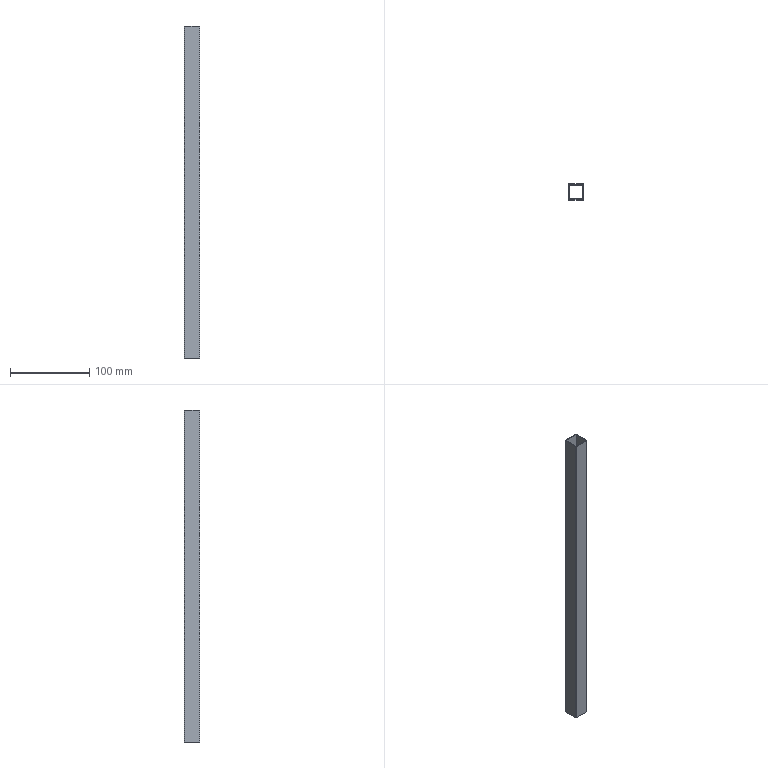Component | SolidWorks | Drawer_Rib-1 | 1 solid | 14 faces | box 20 x 20 x 420 mm | volume 37540 mm3 | plane 10 | cylinder 4 | commonest cylinder face diameters 2 x4
build123d program:
from build123d import *

# Parameters (mm, degrees)
SKETCH1_W           = 17.6
SKETCH1_H           = 17.6
BOSS_EXTRUDE1_DEPTH = 420


with BuildPart() as part:
    # Sketch1 → Boss-Extrude1 (new body)
    with BuildSketch(Plane(origin=(0, 0, 0), x_dir=(1, 0, 0), z_dir=(0, 1, 0))):
        with BuildLine():
            Line((-9, 10), (9, 10))
            ThreePointArc((9, 10), (9.707, 9.707), (10, 9))
            Line((10, 9), (10, -9))
            ThreePointArc((10, -9), (9.707, -9.707), (9, -10))
            Line((9, -10), (-9, -10))
            ThreePointArc((-9, -10), (-9.707, -9.707), (-10, -9))
            Line((-10, -9), (-10, 9))
            ThreePointArc((-10, 9), (-9.707, 9.707), (-9, 10))
        make_face()
        Rectangle(SKETCH1_W, SKETCH1_H, mode=Mode.SUBTRACT)
    extrude(amount=BOSS_EXTRUDE1_DEPTH)


solid = part.part

# Placed as in the assembly
solid = solid.moved(Location((8.5, 246, -100), (90, 0, 0)))
STEP:
#1=COLOUR_RGB('',0.7922,0.8196,0.9333);
#2=FILL_AREA_STYLE_COLOUR('',#1);
#3=FILL_AREA_STYLE('',(#2));
#4=SURFACE_STYLE_FILL_AREA(#3);
#5=SURFACE_SIDE_STYLE('',(#4));
#6=SURFACE_STYLE_USAGE(.BOTH.,#5);
#7=PRESENTATION_STYLE_ASSIGNMENT((#6));
#8=CARTESIAN_POINT('',(-0.01969,9.291,-3.937));
#9=VERTEX_POINT('',#8);
#10=CARTESIAN_POINT('',(-0.05906,9.331,-3.937));
#11=VERTEX_POINT('',#10);
#12=CARTESIAN_POINT('',(-0.01969,9.331,-3.937));
#13=DIRECTION('',(0.,-0.,-1.));
#14=DIRECTION('',(-1.,0.,0.));
#15=AXIS2_PLACEMENT_3D('',#12,#13,#14);
#16=CIRCLE('',#15,0.03937);
#17=EDGE_CURVE('',#9,#11,#16,.T.);
#18=ORIENTED_EDGE('',*,*,#17,.T.);
#19=CARTESIAN_POINT('',(-0.05906,10.039,-3.937));
#20=VERTEX_POINT('',#19);
#21=CARTESIAN_POINT('',(-0.05906,9.331,-3.937));
#22=DIRECTION('',(-0.,1.,-0.));
#23=VECTOR('',#22,39.37);
#24=LINE('',#21,#23);
#25=EDGE_CURVE('',#11,#20,#24,.T.);
#26=ORIENTED_EDGE('',*,*,#25,.T.);
#27=CARTESIAN_POINT('',(-0.01969,10.079,-3.937));
#28=VERTEX_POINT('',#27);
#29=CARTESIAN_POINT('',(-0.01969,10.039,-3.937));
#30=DIRECTION('',(0.,-0.,-1.));
#31=DIRECTION('',(1.,0.,0.));
#32=AXIS2_PLACEMENT_3D('',#29,#30,#31);
#33=CIRCLE('',#32,0.03937);
#34=EDGE_CURVE('',#20,#28,#33,.T.);
#35=ORIENTED_EDGE('',*,*,#34,.T.);
#36=CARTESIAN_POINT('',(0.689,10.079,-3.937));
#37=VERTEX_POINT('',#36);
#38=CARTESIAN_POINT('',(0.689,10.079,-3.937));
#39=DIRECTION('',(1.,-0.,0.));
#40=VECTOR('',#39,39.37);
#41=LINE('',#38,#40);
#42=EDGE_CURVE('',#28,#37,#41,.T.);
#43=ORIENTED_EDGE('',*,*,#42,.T.);
#44=CARTESIAN_POINT('',(0.7283,10.039,-3.937));
#45=VERTEX_POINT('',#44);
#46=CARTESIAN_POINT('',(0.689,10.039,-3.937));
#47=DIRECTION('',(0.,-0.,-1.));
#48=DIRECTION('',(-1.,0.,0.));
#49=AXIS2_PLACEMENT_3D('',#46,#47,#48);
#50=CIRCLE('',#49,0.03937);
#51=EDGE_CURVE('',#37,#45,#50,.T.);
#52=ORIENTED_EDGE('',*,*,#51,.T.);
#53=CARTESIAN_POINT('',(0.7283,9.331,-3.937));
#54=VERTEX_POINT('',#53);
#55=CARTESIAN_POINT('',(0.7283,9.331,-3.937));
#56=DIRECTION('',(0.,-1.,0.));
#57=VECTOR('',#56,39.37);
#58=LINE('',#55,#57);
#59=EDGE_CURVE('',#45,#54,#58,.T.);
#60=ORIENTED_EDGE('',*,*,#59,.T.);
#61=CARTESIAN_POINT('',(0.689,9.291,-3.937));
#62=VERTEX_POINT('',#61);
#63=CARTESIAN_POINT('',(0.689,9.331,-3.937));
#64=DIRECTION('',(0.,-0.,-1.));
#65=DIRECTION('',(-1.,0.,0.));
#66=AXIS2_PLACEMENT_3D('',#63,#64,#65);
#67=CIRCLE('',#66,0.03937);
#68=EDGE_CURVE('',#54,#62,#67,.T.);
#69=ORIENTED_EDGE('',*,*,#68,.T.);
#70=CARTESIAN_POINT('',(0.689,9.291,-3.937));
#71=DIRECTION('',(-1.,0.,-0.));
#72=VECTOR('',#71,39.37);
#73=LINE('',#70,#72);
#74=EDGE_CURVE('',#62,#9,#73,.T.);
#75=ORIENTED_EDGE('',*,*,#74,.T.);
#76=EDGE_LOOP('',(#18,#26,#35,#43,#52,#60,#69,#75));
#77=FACE_OUTER_BOUND('',#76,.T.);
#78=CARTESIAN_POINT('',(0.6811,9.339,-3.937));
#79=VERTEX_POINT('',#78);
#80=CARTESIAN_POINT('',(-0.01181,9.339,-3.937));
#81=VERTEX_POINT('',#80);
#82=CARTESIAN_POINT('',(0.6811,9.339,-3.937));
#83=DIRECTION('',(-1.,-0.,-0.));
#84=VECTOR('',#83,39.37);
#85=LINE('',#82,#84);
#86=EDGE_CURVE('',#79,#81,#85,.T.);
#87=ORIENTED_EDGE('',*,*,#86,.F.);
#88=CARTESIAN_POINT('',(0.6811,10.031,-3.937));
#89=VERTEX_POINT('',#88);
#90=CARTESIAN_POINT('',(0.6811,9.339,-3.937));
#91=DIRECTION('',(0.,-1.,0.));
#92=VECTOR('',#91,39.37);
#93=LINE('',#90,#92);
#94=EDGE_CURVE('',#89,#79,#93,.T.);
#95=ORIENTED_EDGE('',*,*,#94,.F.);
#96=CARTESIAN_POINT('',(-0.01181,10.031,-3.937));
#97=VERTEX_POINT('',#96);
#98=CARTESIAN_POINT('',(0.6811,10.031,-3.937));
#99=DIRECTION('',(1.,0.,0.));
#100=VECTOR('',#99,39.37);
#101=LINE('',#98,#100);
#102=EDGE_CURVE('',#97,#89,#101,.T.);
#103=ORIENTED_EDGE('',*,*,#102,.F.);
#104=CARTESIAN_POINT('',(-0.01181,9.339,-3.937));
#105=DIRECTION('',(-0.,1.,-0.));
#106=VECTOR('',#105,39.37);
#107=LINE('',#104,#106);
#108=EDGE_CURVE('',#81,#97,#107,.T.);
#109=ORIENTED_EDGE('',*,*,#108,.F.);
#110=EDGE_LOOP('',(#87,#95,#103,#109));
#111=FACE_BOUND('',#110,.T.);
#112=CARTESIAN_POINT('',(-0.01969,9.331,-3.937));
#113=DIRECTION('',(0.,-0.,-1.));
#114=DIRECTION('',(-1.,-0.,-0.));
#115=AXIS2_PLACEMENT_3D('',#112,#113,#114);
#116=PLANE('',#115);
#117=ADVANCED_FACE('',(#77,#111),#116,.T.);
#118=CARTESIAN_POINT('',(-0.01969,9.291,12.598));
#119=VERTEX_POINT('',#118);
#120=CARTESIAN_POINT('',(-0.05906,9.331,12.598));
#121=VERTEX_POINT('',#120);
#122=CARTESIAN_POINT('',(-0.01969,9.331,12.598));
#123=DIRECTION('',(0.,-0.,-1.));
#124=DIRECTION('',(-1.,0.,0.));
#125=AXIS2_PLACEMENT_3D('',#122,#123,#124);
#126=CIRCLE('',#125,0.03937);
#127=EDGE_CURVE('',#119,#121,#126,.T.);
#128=ORIENTED_EDGE('',*,*,#127,.F.);
#129=CARTESIAN_POINT('',(0.689,9.291,12.598));
#130=VERTEX_POINT('',#129);
#131=CARTESIAN_POINT('',(0.689,9.291,12.598));
#132=DIRECTION('',(-1.,0.,-0.));
#133=VECTOR('',#132,39.37);
#134=LINE('',#131,#133);
#135=EDGE_CURVE('',#130,#119,#134,.T.);
#136=ORIENTED_EDGE('',*,*,#135,.F.);
#137=CARTESIAN_POINT('',(0.7283,9.331,12.598));
#138=VERTEX_POINT('',#137);
#139=CARTESIAN_POINT('',(0.689,9.331,12.598));
#140=DIRECTION('',(0.,-0.,-1.));
#141=DIRECTION('',(-1.,0.,0.));
#142=AXIS2_PLACEMENT_3D('',#139,#140,#141);
#143=CIRCLE('',#142,0.03937);
#144=EDGE_CURVE('',#138,#130,#143,.T.);
#145=ORIENTED_EDGE('',*,*,#144,.F.);
#146=CARTESIAN_POINT('',(0.7283,10.039,12.598));
#147=VERTEX_POINT('',#146);
#148=CARTESIAN_POINT('',(0.7283,9.331,12.598));
#149=DIRECTION('',(0.,-1.,0.));
#150=VECTOR('',#149,39.37);
#151=LINE('',#148,#150);
#152=EDGE_CURVE('',#147,#138,#151,.T.);
#153=ORIENTED_EDGE('',*,*,#152,.F.);
#154=CARTESIAN_POINT('',(0.689,10.079,12.598));
#155=VERTEX_POINT('',#154);
#156=CARTESIAN_POINT('',(0.689,10.039,12.598));
#157=DIRECTION('',(0.,-0.,-1.));
#158=DIRECTION('',(-1.,0.,0.));
#159=AXIS2_PLACEMENT_3D('',#156,#157,#158);
#160=CIRCLE('',#159,0.03937);
#161=EDGE_CURVE('',#155,#147,#160,.T.);
#162=ORIENTED_EDGE('',*,*,#161,.F.);
#163=CARTESIAN_POINT('',(-0.01969,10.079,12.598));
#164=VERTEX_POINT('',#163);
#165=CARTESIAN_POINT('',(0.689,10.079,12.598));
#166=DIRECTION('',(1.,-0.,0.));
#167=VECTOR('',#166,39.37);
#168=LINE('',#165,#167);
#169=EDGE_CURVE('',#164,#155,#168,.T.);
#170=ORIENTED_EDGE('',*,*,#169,.F.);
#171=CARTESIAN_POINT('',(-0.05906,10.039,12.598));
#172=VERTEX_POINT('',#171);
#173=CARTESIAN_POINT('',(-0.01969,10.039,12.598));
#174=DIRECTION('',(0.,-0.,-1.));
#175=DIRECTION('',(1.,0.,0.));
#176=AXIS2_PLACEMENT_3D('',#173,#174,#175);
#177=CIRCLE('',#176,0.03937);
#178=EDGE_CURVE('',#172,#164,#177,.T.);
#179=ORIENTED_EDGE('',*,*,#178,.F.);
#180=CARTESIAN_POINT('',(-0.05906,9.331,12.598));
#181=DIRECTION('',(-0.,1.,-0.));
#182=VECTOR('',#181,39.37);
#183=LINE('',#180,#182);
#184=EDGE_CURVE('',#121,#172,#183,.T.);
#185=ORIENTED_EDGE('',*,*,#184,.F.);
#186=EDGE_LOOP('',(#128,#136,#145,#153,#162,#170,#179,#185));
#187=FACE_OUTER_BOUND('',#186,.T.);
#188=CARTESIAN_POINT('',(0.6811,10.031,12.598));
#189=VERTEX_POINT('',#188);
#190=CARTESIAN_POINT('',(0.6811,9.339,12.598));
#191=VERTEX_POINT('',#190);
#192=CARTESIAN_POINT('',(0.6811,9.339,12.598));
#193=DIRECTION('',(0.,-1.,0.));
#194=VECTOR('',#193,39.37);
#195=LINE('',#192,#194);
#196=EDGE_CURVE('',#189,#191,#195,.T.);
#197=ORIENTED_EDGE('',*,*,#196,.T.);
#198=CARTESIAN_POINT('',(-0.01181,9.339,12.598));
#199=VERTEX_POINT('',#198);
#200=CARTESIAN_POINT('',(0.6811,9.339,12.598));
#201=DIRECTION('',(-1.,-0.,-0.));
#202=VECTOR('',#201,39.37);
#203=LINE('',#200,#202);
#204=EDGE_CURVE('',#191,#199,#203,.T.);
#205=ORIENTED_EDGE('',*,*,#204,.T.);
#206=CARTESIAN_POINT('',(-0.01181,10.031,12.598));
#207=VERTEX_POINT('',#206);
#208=CARTESIAN_POINT('',(-0.01181,9.339,12.598));
#209=DIRECTION('',(-0.,1.,-0.));
#210=VECTOR('',#209,39.37);
#211=LINE('',#208,#210);
#212=EDGE_CURVE('',#199,#207,#211,.T.);
#213=ORIENTED_EDGE('',*,*,#212,.T.);
#214=CARTESIAN_POINT('',(0.6811,10.031,12.598));
#215=DIRECTION('',(1.,0.,0.));
#216=VECTOR('',#215,39.37);
#217=LINE('',#214,#216);
#218=EDGE_CURVE('',#207,#189,#217,.T.);
#219=ORIENTED_EDGE('',*,*,#218,.T.);
#220=EDGE_LOOP('',(#197,#205,#213,#219));
#221=FACE_BOUND('',#220,.T.);
#222=CARTESIAN_POINT('',(-0.01969,9.331,12.598));
#223=DIRECTION('',(0.,-0.,-1.));
#224=DIRECTION('',(-1.,-0.,-0.));
#225=AXIS2_PLACEMENT_3D('',#222,#223,#224);
#226=PLANE('',#225);
#227=ADVANCED_FACE('',(#187,#221),#226,.F.);
#228=ORIENTED_EDGE('',*,*,#127,.T.);
#229=CARTESIAN_POINT('',(-0.05906,9.331,-3.937));
#230=DIRECTION('',(-0.,0.,1.));
#231=VECTOR('',#230,39.37);
#232=LINE('',#229,#231);
#233=EDGE_CURVE('',#11,#121,#232,.T.);
#234=ORIENTED_EDGE('',*,*,#233,.F.);
#235=ORIENTED_EDGE('',*,*,#17,.F.);
#236=CARTESIAN_POINT('',(-0.01969,9.291,-3.937));
#237=DIRECTION('',(-0.,0.,1.));
#238=VECTOR('',#237,39.37);
#239=LINE('',#236,#238);
#240=EDGE_CURVE('',#9,#119,#239,.T.);
#241=ORIENTED_EDGE('',*,*,#240,.T.);
#242=EDGE_LOOP('',(#228,#234,#235,#241));
#243=FACE_OUTER_BOUND('',#242,.T.);
#244=CARTESIAN_POINT('',(-0.01969,9.331,-3.937));
#245=DIRECTION('',(-0.,0.,1.));
#246=DIRECTION('',(1.,0.,0.));
#247=AXIS2_PLACEMENT_3D('',#244,#245,#246);
#248=CYLINDRICAL_SURFACE('',#247,0.03937);
#249=ADVANCED_FACE('',(#243),#248,.T.);
#250=ORIENTED_EDGE('',*,*,#184,.T.);
#251=CARTESIAN_POINT('',(-0.05906,10.039,-3.937));
#252=DIRECTION('',(-0.,0.,1.));
#253=VECTOR('',#252,39.37);
#254=LINE('',#251,#253);
#255=EDGE_CURVE('',#20,#172,#254,.T.);
#256=ORIENTED_EDGE('',*,*,#255,.F.);
#257=ORIENTED_EDGE('',*,*,#25,.F.);
#258=ORIENTED_EDGE('',*,*,#233,.T.);
#259=EDGE_LOOP('',(#250,#256,#257,#258));
#260=FACE_OUTER_BOUND('',#259,.T.);
#261=CARTESIAN_POINT('',(-0.05906,9.331,-3.937));
#262=DIRECTION('',(1.,0.,0.));
#263=DIRECTION('',(0.,-1.,0.));
#264=AXIS2_PLACEMENT_3D('',#261,#262,#263);
#265=PLANE('',#264);
#266=ADVANCED_FACE('',(#260),#265,.F.);
#267=ORIENTED_EDGE('',*,*,#178,.T.);
#268=CARTESIAN_POINT('',(-0.01969,10.079,-3.937));
#269=DIRECTION('',(-0.,0.,1.));
#270=VECTOR('',#269,39.37);
#271=LINE('',#268,#270);
#272=EDGE_CURVE('',#28,#164,#271,.T.);
#273=ORIENTED_EDGE('',*,*,#272,.F.);
#274=ORIENTED_EDGE('',*,*,#34,.F.);
#275=ORIENTED_EDGE('',*,*,#255,.T.);
#276=EDGE_LOOP('',(#267,#273,#274,#275));
#277=FACE_OUTER_BOUND('',#276,.T.);
#278=CARTESIAN_POINT('',(-0.01969,10.039,-3.937));
#279=DIRECTION('',(-0.,0.,1.));
#280=DIRECTION('',(1.,0.,0.));
#281=AXIS2_PLACEMENT_3D('',#278,#279,#280);
#282=CYLINDRICAL_SURFACE('',#281,0.03937);
#283=ADVANCED_FACE('',(#277),#282,.T.);
#284=ORIENTED_EDGE('',*,*,#169,.T.);
#285=CARTESIAN_POINT('',(0.689,10.079,-3.937));
#286=DIRECTION('',(-0.,0.,1.));
#287=VECTOR('',#286,39.37);
#288=LINE('',#285,#287);
#289=EDGE_CURVE('',#37,#155,#288,.T.);
#290=ORIENTED_EDGE('',*,*,#289,.F.);
#291=ORIENTED_EDGE('',*,*,#42,.F.);
#292=ORIENTED_EDGE('',*,*,#272,.T.);
#293=EDGE_LOOP('',(#284,#290,#291,#292));
#294=FACE_OUTER_BOUND('',#293,.T.);
#295=CARTESIAN_POINT('',(0.689,10.079,-3.937));
#296=DIRECTION('',(-0.,-1.,0.));
#297=DIRECTION('',(-1.,0.,-0.));
#298=AXIS2_PLACEMENT_3D('',#295,#296,#297);
#299=PLANE('',#298);
#300=ADVANCED_FACE('',(#294),#299,.F.);
#301=ORIENTED_EDGE('',*,*,#161,.T.);
#302=CARTESIAN_POINT('',(0.7283,10.039,-3.937));
#303=DIRECTION('',(-0.,0.,1.));
#304=VECTOR('',#303,39.37);
#305=LINE('',#302,#304);
#306=EDGE_CURVE('',#45,#147,#305,.T.);
#307=ORIENTED_EDGE('',*,*,#306,.F.);
#308=ORIENTED_EDGE('',*,*,#51,.F.);
#309=ORIENTED_EDGE('',*,*,#289,.T.);
#310=EDGE_LOOP('',(#301,#307,#308,#309));
#311=FACE_OUTER_BOUND('',#310,.T.);
#312=CARTESIAN_POINT('',(0.689,10.039,-3.937));
#313=DIRECTION('',(-0.,0.,1.));
#314=DIRECTION('',(1.,0.,0.));
#315=AXIS2_PLACEMENT_3D('',#312,#313,#314);
#316=CYLINDRICAL_SURFACE('',#315,0.03937);
#317=ADVANCED_FACE('',(#311),#316,.T.);
#318=ORIENTED_EDGE('',*,*,#152,.T.);
#319=CARTESIAN_POINT('',(0.7283,9.331,-3.937));
#320=DIRECTION('',(-0.,0.,1.));
#321=VECTOR('',#320,39.37);
#322=LINE('',#319,#321);
#323=EDGE_CURVE('',#54,#138,#322,.T.);
#324=ORIENTED_EDGE('',*,*,#323,.F.);
#325=ORIENTED_EDGE('',*,*,#59,.F.);
#326=ORIENTED_EDGE('',*,*,#306,.T.);
#327=EDGE_LOOP('',(#318,#324,#325,#326));
#328=FACE_OUTER_BOUND('',#327,.T.);
#329=CARTESIAN_POINT('',(0.7283,9.331,-3.937));
#330=DIRECTION('',(-1.,-0.,-0.));
#331=DIRECTION('',(-0.,1.,-0.));
#332=AXIS2_PLACEMENT_3D('',#329,#330,#331);
#333=PLANE('',#332);
#334=ADVANCED_FACE('',(#328),#333,.F.);
#335=ORIENTED_EDGE('',*,*,#144,.T.);
#336=CARTESIAN_POINT('',(0.689,9.291,-3.937));
#337=DIRECTION('',(-0.,0.,1.));
#338=VECTOR('',#337,39.37);
#339=LINE('',#336,#338);
#340=EDGE_CURVE('',#62,#130,#339,.T.);
#341=ORIENTED_EDGE('',*,*,#340,.F.);
#342=ORIENTED_EDGE('',*,*,#68,.F.);
#343=ORIENTED_EDGE('',*,*,#323,.T.);
#344=EDGE_LOOP('',(#335,#341,#342,#343));
#345=FACE_OUTER_BOUND('',#344,.T.);
#346=CARTESIAN_POINT('',(0.689,9.331,-3.937));
#347=DIRECTION('',(-0.,0.,1.));
#348=DIRECTION('',(1.,0.,0.));
#349=AXIS2_PLACEMENT_3D('',#346,#347,#348);
#350=CYLINDRICAL_SURFACE('',#349,0.03937);
#351=ADVANCED_FACE('',(#345),#350,.T.);
#352=ORIENTED_EDGE('',*,*,#135,.T.);
#353=ORIENTED_EDGE('',*,*,#240,.F.);
#354=ORIENTED_EDGE('',*,*,#74,.F.);
#355=ORIENTED_EDGE('',*,*,#340,.T.);
#356=EDGE_LOOP('',(#352,#353,#354,#355));
#357=FACE_OUTER_BOUND('',#356,.T.);
#358=CARTESIAN_POINT('',(0.689,9.291,-3.937));
#359=DIRECTION('',(0.,1.,-0.));
#360=DIRECTION('',(1.,-0.,0.));
#361=AXIS2_PLACEMENT_3D('',#358,#359,#360);
#362=PLANE('',#361);
#363=ADVANCED_FACE('',(#357),#362,.F.);
#364=ORIENTED_EDGE('',*,*,#196,.F.);
#365=CARTESIAN_POINT('',(0.6811,10.031,-3.937));
#366=DIRECTION('',(-0.,0.,1.));
#367=VECTOR('',#366,39.37);
#368=LINE('',#365,#367);
#369=EDGE_CURVE('',#89,#189,#368,.T.);
#370=ORIENTED_EDGE('',*,*,#369,.F.);
#371=ORIENTED_EDGE('',*,*,#94,.T.);
#372=CARTESIAN_POINT('',(0.6811,9.339,-3.937));
#373=DIRECTION('',(-0.,0.,1.));
#374=VECTOR('',#373,39.37);
#375=LINE('',#372,#374);
#376=EDGE_CURVE('',#79,#191,#375,.T.);
#377=ORIENTED_EDGE('',*,*,#376,.T.);
#378=EDGE_LOOP('',(#364,#370,#371,#377));
#379=FACE_OUTER_BOUND('',#378,.T.);
#380=CARTESIAN_POINT('',(0.6811,9.339,-3.937));
#381=DIRECTION('',(-1.,-0.,-0.));
#382=DIRECTION('',(-0.,1.,-0.));
#383=AXIS2_PLACEMENT_3D('',#380,#381,#382);
#384=PLANE('',#383);
#385=ADVANCED_FACE('',(#379),#384,.T.);
#386=ORIENTED_EDGE('',*,*,#204,.F.);
#387=ORIENTED_EDGE('',*,*,#376,.F.);
#388=ORIENTED_EDGE('',*,*,#86,.T.);
#389=CARTESIAN_POINT('',(-0.01181,9.339,-3.937));
#390=DIRECTION('',(-0.,0.,1.));
#391=VECTOR('',#390,39.37);
#392=LINE('',#389,#391);
#393=EDGE_CURVE('',#81,#199,#392,.T.);
#394=ORIENTED_EDGE('',*,*,#393,.T.);
#395=EDGE_LOOP('',(#386,#387,#388,#394));
#396=FACE_OUTER_BOUND('',#395,.T.);
#397=CARTESIAN_POINT('',(0.6811,9.339,-3.937));
#398=DIRECTION('',(-0.,1.,-0.));
#399=DIRECTION('',(1.,0.,0.));
#400=AXIS2_PLACEMENT_3D('',#397,#398,#399);
#401=PLANE('',#400);
#402=ADVANCED_FACE('',(#396),#401,.T.);
#403=ORIENTED_EDGE('',*,*,#212,.F.);
#404=ORIENTED_EDGE('',*,*,#393,.F.);
#405=ORIENTED_EDGE('',*,*,#108,.T.);
#406=CARTESIAN_POINT('',(-0.01181,10.031,-3.937));
#407=DIRECTION('',(-0.,0.,1.));
#408=VECTOR('',#407,39.37);
#409=LINE('',#406,#408);
#410=EDGE_CURVE('',#97,#207,#409,.T.);
#411=ORIENTED_EDGE('',*,*,#410,.T.);
#412=EDGE_LOOP('',(#403,#404,#405,#411));
#413=FACE_OUTER_BOUND('',#412,.T.);
#414=CARTESIAN_POINT('',(-0.01181,9.339,-3.937));
#415=DIRECTION('',(1.,0.,0.));
#416=DIRECTION('',(0.,-1.,0.));
#417=AXIS2_PLACEMENT_3D('',#414,#415,#416);
#418=PLANE('',#417);
#419=ADVANCED_FACE('',(#413),#418,.T.);
#420=ORIENTED_EDGE('',*,*,#218,.F.);
#421=ORIENTED_EDGE('',*,*,#410,.F.);
#422=ORIENTED_EDGE('',*,*,#102,.T.);
#423=ORIENTED_EDGE('',*,*,#369,.T.);
#424=EDGE_LOOP('',(#420,#421,#422,#423));
#425=FACE_OUTER_BOUND('',#424,.T.);
#426=CARTESIAN_POINT('',(0.6811,10.031,-3.937));
#427=DIRECTION('',(0.,-1.,0.));
#428=DIRECTION('',(-1.,-0.,-0.));
#429=AXIS2_PLACEMENT_3D('',#426,#427,#428);
#430=PLANE('',#429);
#431=ADVANCED_FACE('',(#425),#430,.T.);
#432=CLOSED_SHELL('',(#117,#227,#249,#266,#283,#300,#317,#334,#351,#363,#385,#402,#419,#431));
#433=MANIFOLD_SOLID_BREP('',#432);
#434=STYLED_ITEM('',(#7),#433);
#435=(LENGTH_UNIT()NAMED_UNIT(*)SI_UNIT($,.METRE.));
#436=LENGTH_MEASURE_WITH_UNIT(LENGTH_MEASURE(0.0254),#435);
#437=DIMENSIONAL_EXPONENTS(1.,0.,0.,0.,0.,0.,0.);
#438=(CONVERSION_BASED_UNIT('',#436)LENGTH_UNIT()NAMED_UNIT(#437));
#439=UNCERTAINTY_MEASURE_WITH_UNIT(LENGTH_MEASURE(0.00001),#438,'','');
#440=(NAMED_UNIT(*)PLANE_ANGLE_UNIT()SI_UNIT($,.RADIAN.));
#441=(NAMED_UNIT(*)SI_UNIT($,.STERADIAN.)SOLID_ANGLE_UNIT());
#442=(GEOMETRIC_REPRESENTATION_CONTEXT(3)GLOBAL_UNCERTAINTY_ASSIGNED_CONTEXT((#439))GLOBAL_UNIT_ASSIGNED_CONTEXT((#438,#440,#441))REPRESENTATION_CONTEXT('',''));
#443=MECHANICAL_DESIGN_GEOMETRIC_PRESENTATION_REPRESENTATION('',(#434),#442);
#444=CARTESIAN_POINT('',(0.,0.,0.));
#445=DIRECTION('',(0.,0.,1.));
#446=DIRECTION('',(1.,0.,0.));
#447=AXIS2_PLACEMENT_3D('',#444,#445,#446);
#448=(LENGTH_UNIT()NAMED_UNIT(*)SI_UNIT($,.METRE.));
#449=LENGTH_MEASURE_WITH_UNIT(LENGTH_MEASURE(0.0254),#448);
#450=DIMENSIONAL_EXPONENTS(1.,0.,0.,0.,0.,0.,0.);
#451=(CONVERSION_BASED_UNIT('',#449)LENGTH_UNIT()NAMED_UNIT(#450));
#452=UNCERTAINTY_MEASURE_WITH_UNIT(LENGTH_MEASURE(0.00001),#451,'','');
#453=(NAMED_UNIT(*)PLANE_ANGLE_UNIT()SI_UNIT($,.RADIAN.));
#454=(NAMED_UNIT(*)SI_UNIT($,.STERADIAN.)SOLID_ANGLE_UNIT());
#455=(GEOMETRIC_REPRESENTATION_CONTEXT(3)GLOBAL_UNCERTAINTY_ASSIGNED_CONTEXT((#452))GLOBAL_UNIT_ASSIGNED_CONTEXT((#451,#453,#454))REPRESENTATION_CONTEXT('',''));
#456=ADVANCED_BREP_SHAPE_REPRESENTATION('',(#433,#447),#455);
#457=PRESENTATION_LAYER_ASSIGNMENT('','',(#434));